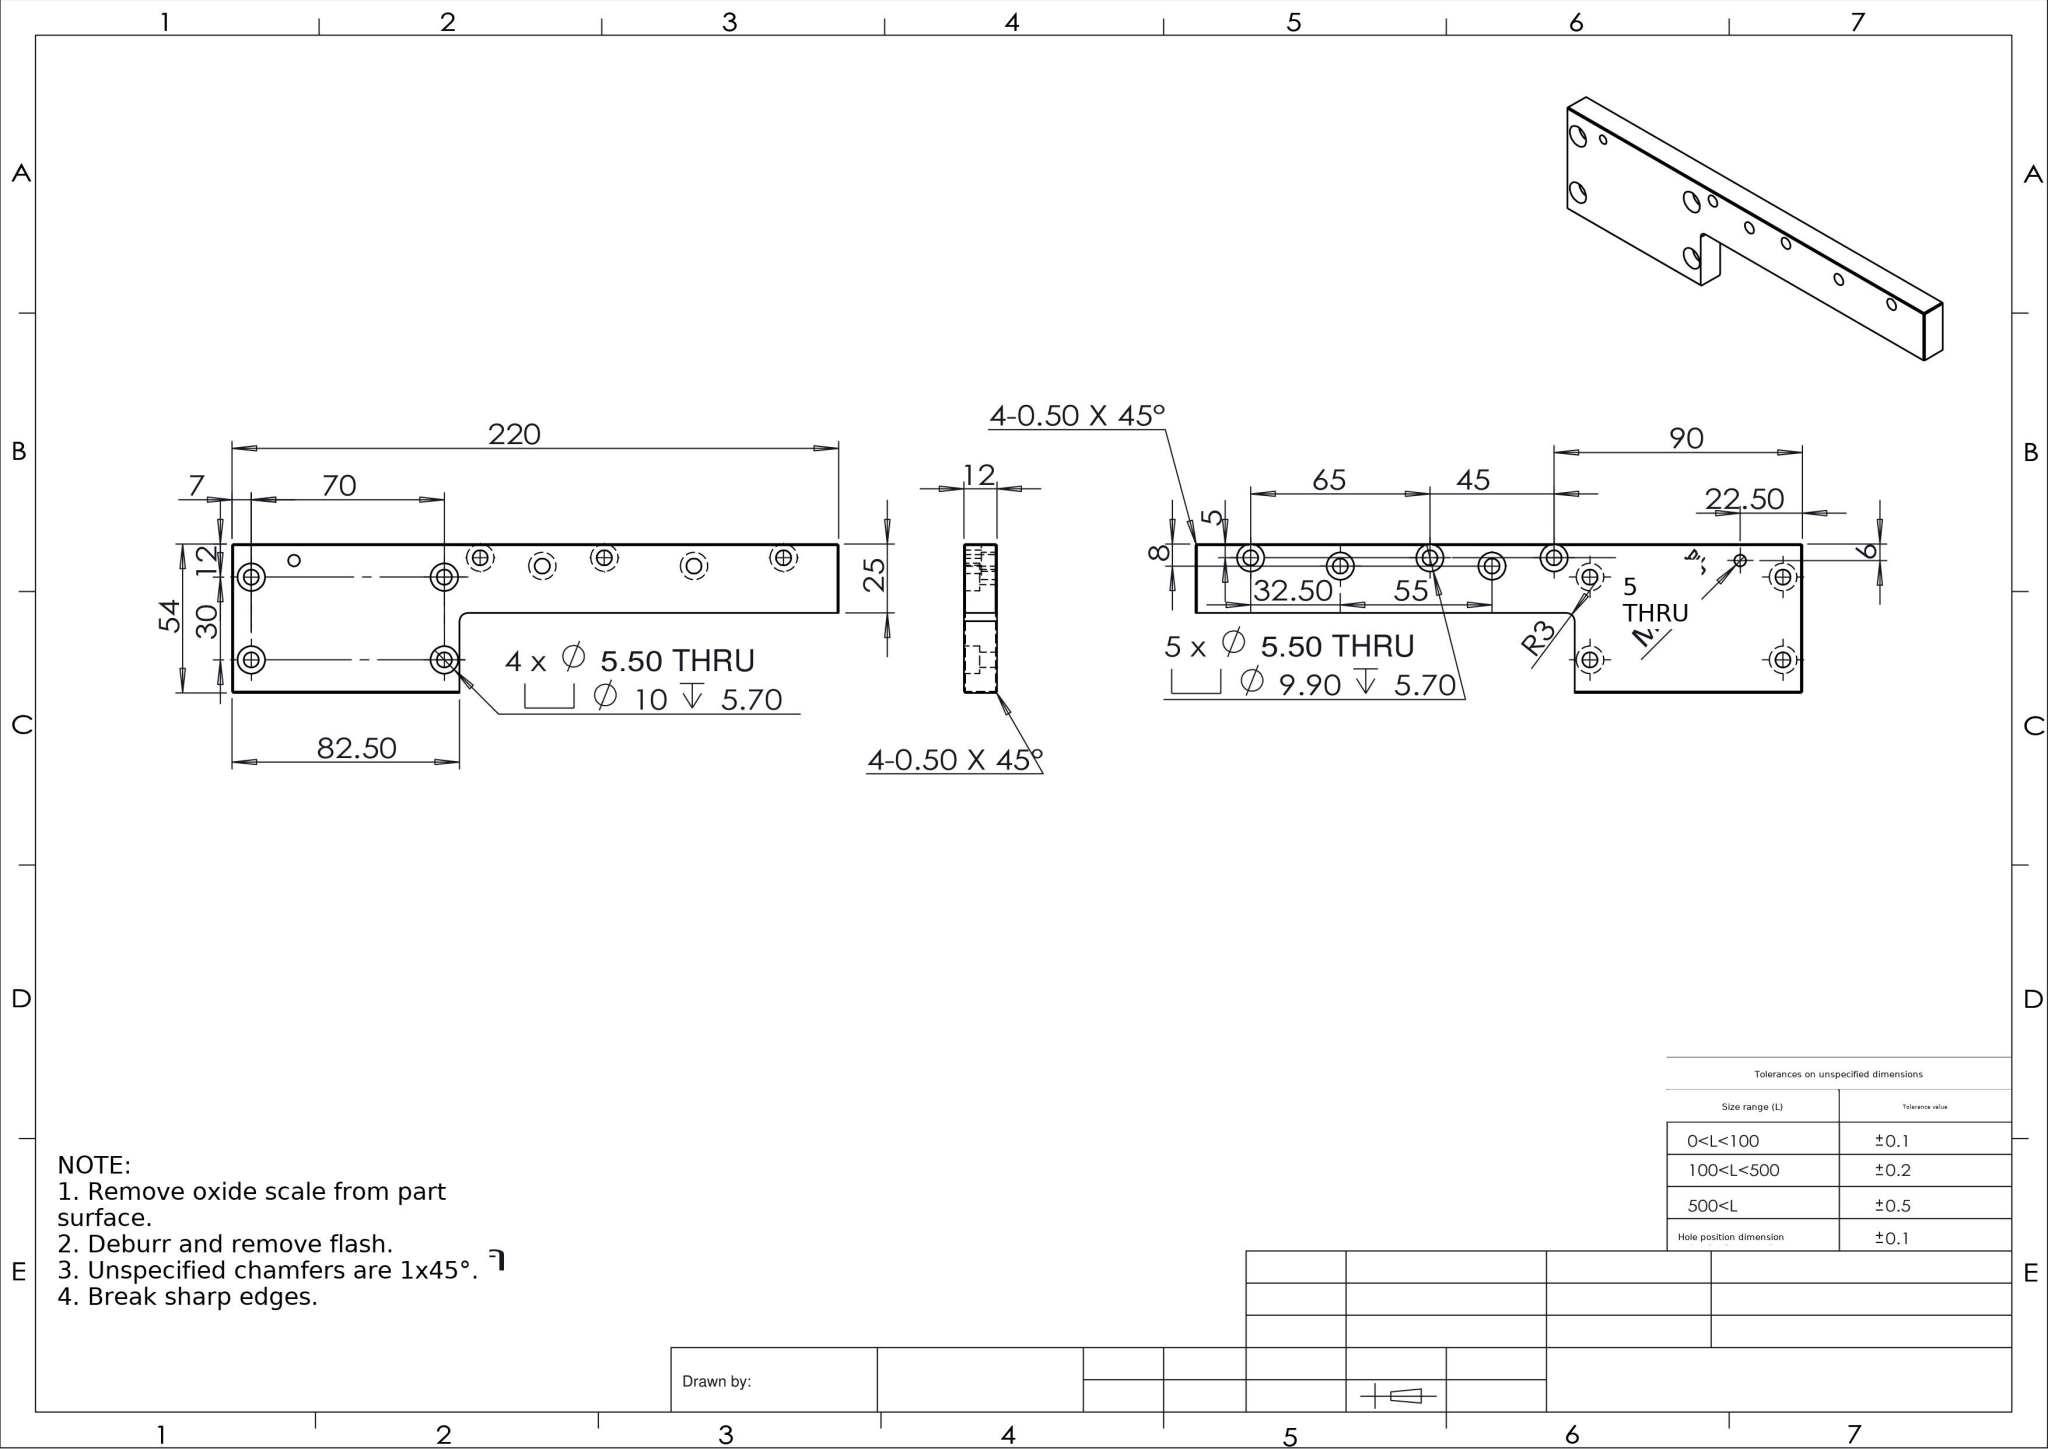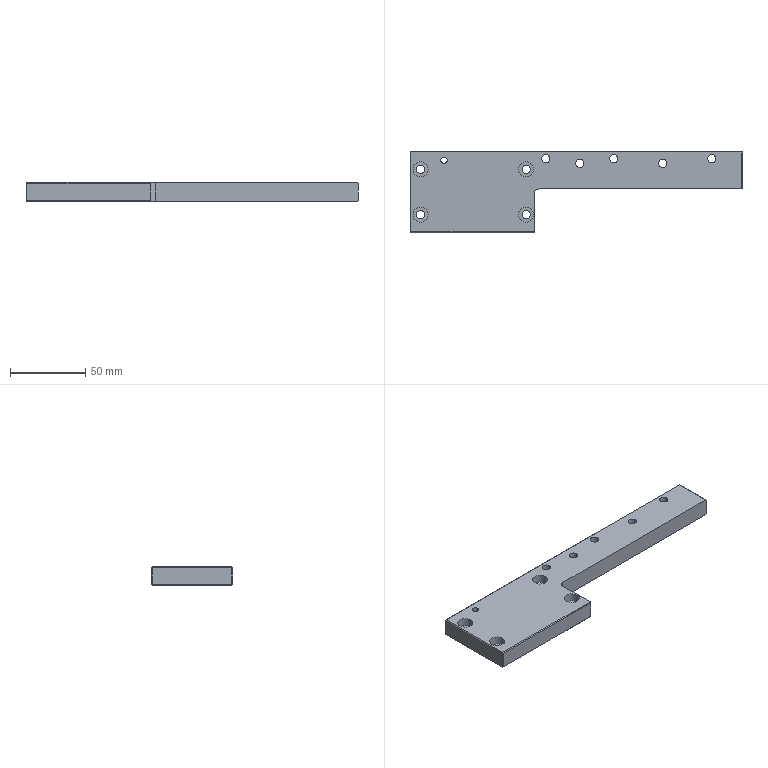Part | SolidWorks | mm | 1 solid | 73 faces | box 220 x 54 x 12 mm | volume 89137 mm3 | cylinder 39 | plane 34 | commonest cylinder face diameters 5.5 x18 9.9 x10 10 x8 4.2 x2 6 x1